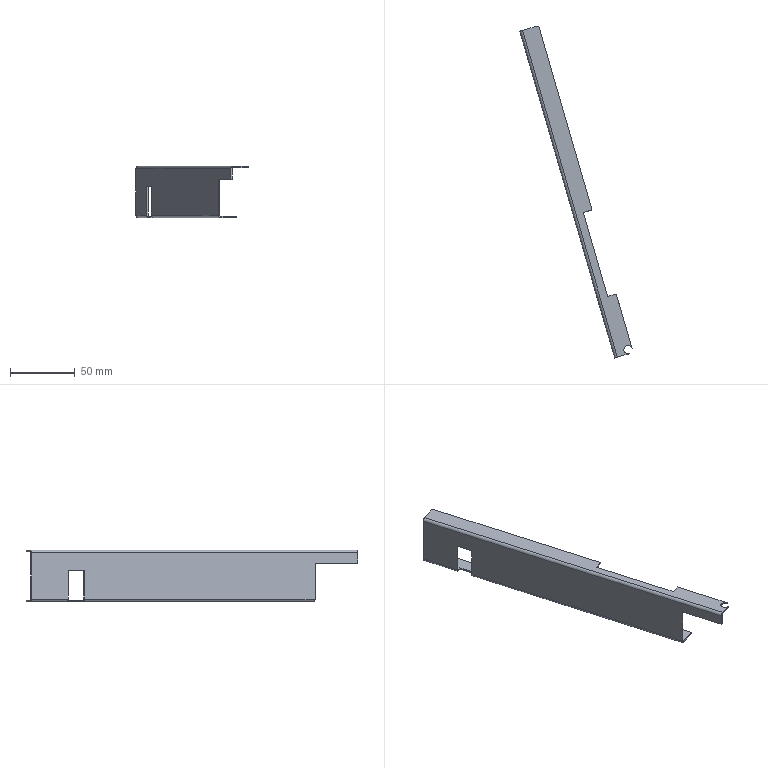Component | SolidWorks | LeftDoorAssembly-1_EndCap1-1 | 1 solid | 39 faces | volume 17476 mm3 | plane 30 | cylinder 9 | commonest cylinder face diameters 2 x5 4.4 x3 6.5 x1